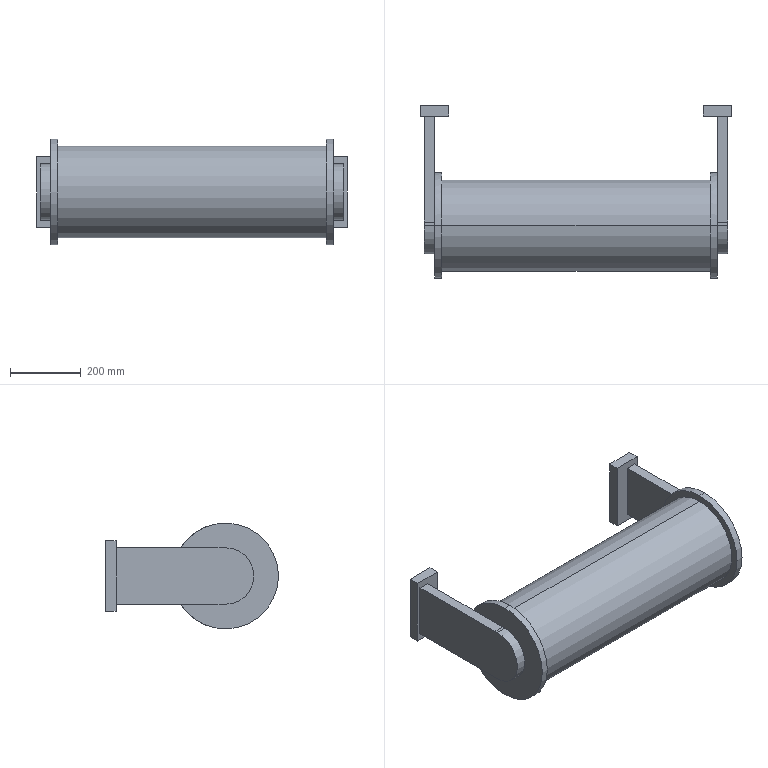Component | SolidWorks | LiftingAndOperatingMechanism-1_22-1 | 1 solid | 36 faces | box 880 x 490 x 300 mm | volume 47705868 mm3 | plane 24 | cylinder 12 | commonest cylinder face diameters 160 x6 300 x4 260 x2
build123d program:
from build123d import *

# Parameters (mm, degrees)
SKETCH3_R           = 150
BOSS_EXTRUDE1_DEPTH = 400
BOSS_EXTRUDE2_DEPTH = 30
SKETCH1_W           = 200
SKETCH1_H           = 80
BOSS_EXTRUDE3_DEPTH = 30
SKETCH5_R           = 150
SKETCH5_R_2         = 130
CUT_EXTRUDE1_DEPTH  = 380


with BuildPart() as part:
    # Sketch3 → Boss-Extrude1 (new, symmetric)
    with BuildSketch(Plane.XY):
        with Locations((0, 310)):
            Circle(SKETCH3_R)
    extrude(amount=BOSS_EXTRUDE1_DEPTH, both=True)

    # Sketch4 → Boss-Extrude2 (add)
    with BuildSketch(Plane.XY.offset(400)):
        with BuildLine():
            Line((-80, 0), (-79.382, 300.077))
            ThreePointArc((-79.382, 300.077), (0, 390), (79.382, 300.077))
            Line((79.382, 300.077), (80, 0))
            Line((80, 0), (-80, 0))
        make_face()
    boss_extrude2 = extrude(amount=BOSS_EXTRUDE2_DEPTH)

    # Mirror1: Boss-Extrude2 across plane
    add(boss_extrude2.mirror(Plane.XY))

    # Sketch1 → Boss-Extrude3 (add)
    with BuildSketch(Plane(origin=(0, 0, 0), x_dir=(1, 0, 0), z_dir=(0, 1, 0))):
        with Locations((0, 400)):
            Rectangle(SKETCH1_W, SKETCH1_H)
        with Locations((0, -400)):
            Rectangle(SKETCH1_W, SKETCH1_H)
    extrude(amount=-BOSS_EXTRUDE3_DEPTH)

    # Sketch5 → Cut-Extrude1 (cut, symmetric)
    with BuildSketch(Plane.XY):
        with Locations(Location((0, 310, 0), (0, 0, 237.939))):
            Circle(SKETCH5_R)
        with Locations((0, 310)):
            Circle(SKETCH5_R_2, mode=Mode.SUBTRACT)
    extrude(amount=CUT_EXTRUDE1_DEPTH, both=True, mode=Mode.SUBTRACT)


solid = part.part

# Placed as in the assembly
solid = solid.moved(Location((-1158.963, 12408.918, 7532.153), (180, 90, 0)))
STEP:
#1=COLOUR_RGB('',0.7922,0.8196,0.9333);
#2=FILL_AREA_STYLE_COLOUR('',#1);
#3=FILL_AREA_STYLE('',(#2));
#4=SURFACE_STYLE_FILL_AREA(#3);
#5=SURFACE_SIDE_STYLE('',(#4));
#6=SURFACE_STYLE_USAGE(.BOTH.,#5);
#7=PRESENTATION_STYLE_ASSIGNMENT((#6));
#8=CARTESIAN_POINT('',(-61.376,476.335,290.636));
#9=VERTEX_POINT('',#8);
#10=CARTESIAN_POINT('',(-61.376,476.335,302.447));
#11=VERTEX_POINT('',#10);
#12=CARTESIAN_POINT('',(-61.376,476.335,296.541));
#13=DIRECTION('',(-1.,-0.,0.0000002));
#14=DIRECTION('',(-0.0000002,0.,-1.));
#15=AXIS2_PLACEMENT_3D('',#12,#13,#14);
#16=CIRCLE('',#15,5.906);
#17=EDGE_CURVE('',#9,#11,#16,.T.);
#18=ORIENTED_EDGE('',*,*,#17,.F.);
#19=CARTESIAN_POINT('',(-60.589,476.335,290.636));
#20=VERTEX_POINT('',#19);
#21=CARTESIAN_POINT('',(-61.376,476.335,290.636));
#22=DIRECTION('',(1.,0.,-0.0000002));
#23=VECTOR('',#22,39.37);
#24=LINE('',#21,#23);
#25=EDGE_CURVE('',#9,#20,#24,.T.);
#26=ORIENTED_EDGE('',*,*,#25,.T.);
#27=CARTESIAN_POINT('',(-60.589,476.335,302.447));
#28=VERTEX_POINT('',#27);
#29=CARTESIAN_POINT('',(-60.589,476.335,296.541));
#30=DIRECTION('',(-1.,-0.,0.0000002));
#31=DIRECTION('',(-0.0000002,0.,-1.));
#32=AXIS2_PLACEMENT_3D('',#29,#30,#31);
#33=CIRCLE('',#32,5.906);
#34=EDGE_CURVE('',#20,#28,#33,.T.);
#35=ORIENTED_EDGE('',*,*,#34,.T.);
#36=CARTESIAN_POINT('',(-61.376,476.335,302.447));
#37=DIRECTION('',(1.,0.,-0.0000002));
#38=VECTOR('',#37,39.37);
#39=LINE('',#36,#38);
#40=EDGE_CURVE('',#11,#28,#39,.T.);
#41=ORIENTED_EDGE('',*,*,#40,.F.);
#42=EDGE_LOOP('',(#18,#26,#35,#41));
#43=FACE_OUTER_BOUND('',#42,.T.);
#44=CARTESIAN_POINT('',(-61.376,476.335,296.541));
#45=DIRECTION('',(1.,0.,-0.0000002));
#46=DIRECTION('',(0.0000002,0.,1.));
#47=AXIS2_PLACEMENT_3D('',#44,#45,#46);
#48=CYLINDRICAL_SURFACE('',#47,5.906);
#49=ADVANCED_FACE('',(#43),#48,.T.);
#50=CARTESIAN_POINT('',(-62.558,476.335,293.392));
#51=VERTEX_POINT('',#50);
#52=CARTESIAN_POINT('',(-62.558,476.335,299.691));
#53=VERTEX_POINT('',#52);
#54=CARTESIAN_POINT('',(-62.558,476.335,296.541));
#55=DIRECTION('',(-1.,-0.,0.0000002));
#56=DIRECTION('',(-0.0000002,0.,-1.));
#57=AXIS2_PLACEMENT_3D('',#54,#55,#56);
#58=CIRCLE('',#57,3.15);
#59=EDGE_CURVE('',#51,#53,#58,.T.);
#60=ORIENTED_EDGE('',*,*,#59,.F.);
#61=CARTESIAN_POINT('',(-61.376,476.335,293.392));
#62=VERTEX_POINT('',#61);
#63=CARTESIAN_POINT('',(-62.558,476.335,293.392));
#64=DIRECTION('',(1.,0.,-0.0000002));
#65=VECTOR('',#64,39.37);
#66=LINE('',#63,#65);
#67=EDGE_CURVE('',#51,#62,#66,.T.);
#68=ORIENTED_EDGE('',*,*,#67,.T.);
#69=CARTESIAN_POINT('',(-61.376,476.335,299.691));
#70=VERTEX_POINT('',#69);
#71=CARTESIAN_POINT('',(-61.376,476.335,296.541));
#72=DIRECTION('',(-1.,-0.,0.0000002));
#73=DIRECTION('',(-0.0000002,0.,-1.));
#74=AXIS2_PLACEMENT_3D('',#71,#72,#73);
#75=CIRCLE('',#74,3.15);
#76=EDGE_CURVE('',#62,#70,#75,.T.);
#77=ORIENTED_EDGE('',*,*,#76,.T.);
#78=CARTESIAN_POINT('',(-62.558,476.335,299.691));
#79=DIRECTION('',(1.,0.,-0.0000002));
#80=VECTOR('',#79,39.37);
#81=LINE('',#78,#80);
#82=EDGE_CURVE('',#53,#70,#81,.T.);
#83=ORIENTED_EDGE('',*,*,#82,.F.);
#84=EDGE_LOOP('',(#60,#68,#77,#83));
#85=FACE_OUTER_BOUND('',#84,.T.);
#86=CARTESIAN_POINT('',(-62.558,476.335,296.541));
#87=DIRECTION('',(1.,0.,-0.0000002));
#88=DIRECTION('',(0.0000002,0.,1.));
#89=AXIS2_PLACEMENT_3D('',#86,#87,#88);
#90=CYLINDRICAL_SURFACE('',#89,3.15);
#91=ADVANCED_FACE('',(#85),#90,.T.);
#92=CARTESIAN_POINT('',(-62.558,476.726,299.667));
#93=VERTEX_POINT('',#92);
#94=CARTESIAN_POINT('',(-62.558,476.335,296.541));
#95=DIRECTION('',(-1.,-0.,0.0000002));
#96=DIRECTION('',(-0.0000002,0.,-1.));
#97=AXIS2_PLACEMENT_3D('',#94,#95,#96);
#98=CIRCLE('',#97,3.15);
#99=EDGE_CURVE('',#53,#93,#98,.T.);
#100=ORIENTED_EDGE('',*,*,#99,.F.);
#101=ORIENTED_EDGE('',*,*,#82,.T.);
#102=CARTESIAN_POINT('',(-61.376,476.726,299.667));
#103=VERTEX_POINT('',#102);
#104=CARTESIAN_POINT('',(-61.376,476.335,296.541));
#105=DIRECTION('',(-1.,-0.,0.0000002));
#106=DIRECTION('',(-0.0000002,0.,-1.));
#107=AXIS2_PLACEMENT_3D('',#104,#105,#106);
#108=CIRCLE('',#107,3.15);
#109=EDGE_CURVE('',#70,#103,#108,.T.);
#110=ORIENTED_EDGE('',*,*,#109,.T.);
#111=CARTESIAN_POINT('',(-62.558,476.726,299.667));
#112=DIRECTION('',(1.,0.,-0.0000002));
#113=VECTOR('',#112,39.37);
#114=LINE('',#111,#113);
#115=EDGE_CURVE('',#93,#103,#114,.T.);
#116=ORIENTED_EDGE('',*,*,#115,.F.);
#117=EDGE_LOOP('',(#100,#101,#110,#116));
#118=FACE_OUTER_BOUND('',#117,.T.);
#119=CARTESIAN_POINT('',(-62.558,476.335,296.541));
#120=DIRECTION('',(1.,0.,-0.0000002));
#121=DIRECTION('',(0.0000002,0.,1.));
#122=AXIS2_PLACEMENT_3D('',#119,#120,#121);
#123=CYLINDRICAL_SURFACE('',#122,3.15);
#124=ADVANCED_FACE('',(#118),#123,.T.);
#125=CARTESIAN_POINT('',(-30.668,476.335,291.423));
#126=VERTEX_POINT('',#125);
#127=CARTESIAN_POINT('',(-30.668,476.335,301.66));
#128=VERTEX_POINT('',#127);
#129=CARTESIAN_POINT('',(-30.668,476.335,296.541));
#130=DIRECTION('',(-1.,-0.,0.0000002));
#131=DIRECTION('',(-0.0000002,0.,-1.));
#132=AXIS2_PLACEMENT_3D('',#129,#130,#131);
#133=CIRCLE('',#132,5.118);
#134=EDGE_CURVE('',#126,#128,#133,.T.);
#135=ORIENTED_EDGE('',*,*,#134,.T.);
#136=CARTESIAN_POINT('',(-60.589,476.335,301.66));
#137=VERTEX_POINT('',#136);
#138=CARTESIAN_POINT('',(-30.668,476.335,301.66));
#139=DIRECTION('',(-1.,-0.,0.0000002));
#140=VECTOR('',#139,39.37);
#141=LINE('',#138,#140);
#142=EDGE_CURVE('',#128,#137,#141,.T.);
#143=ORIENTED_EDGE('',*,*,#142,.T.);
#144=CARTESIAN_POINT('',(-60.589,476.335,291.423));
#145=VERTEX_POINT('',#144);
#146=CARTESIAN_POINT('',(-60.589,476.335,296.541));
#147=DIRECTION('',(-1.,-0.,0.0000002));
#148=DIRECTION('',(-0.0000002,0.,-1.));
#149=AXIS2_PLACEMENT_3D('',#146,#147,#148);
#150=CIRCLE('',#149,5.118);
#151=EDGE_CURVE('',#145,#137,#150,.T.);
#152=ORIENTED_EDGE('',*,*,#151,.F.);
#153=CARTESIAN_POINT('',(-30.668,476.335,291.423));
#154=DIRECTION('',(-1.,-0.,0.0000002));
#155=VECTOR('',#154,39.37);
#156=LINE('',#153,#155);
#157=EDGE_CURVE('',#126,#145,#156,.T.);
#158=ORIENTED_EDGE('',*,*,#157,.F.);
#159=EDGE_LOOP('',(#135,#143,#152,#158));
#160=FACE_OUTER_BOUND('',#159,.T.);
#161=CARTESIAN_POINT('',(-30.668,476.335,296.541));
#162=DIRECTION('',(-1.,-0.,0.0000002));
#163=DIRECTION('',(-0.0000002,0.,-1.));
#164=AXIS2_PLACEMENT_3D('',#161,#162,#163);
#165=CYLINDRICAL_SURFACE('',#164,5.118);
#166=ADVANCED_FACE('',(#160),#165,.T.);
#167=CARTESIAN_POINT('',(-28.699,476.335,293.392));
#168=VERTEX_POINT('',#167);
#169=CARTESIAN_POINT('',(-28.699,476.335,299.691));
#170=VERTEX_POINT('',#169);
#171=CARTESIAN_POINT('',(-28.699,476.335,296.541));
#172=DIRECTION('',(-1.,-0.,0.0000002));
#173=DIRECTION('',(-0.0000002,0.,-1.));
#174=AXIS2_PLACEMENT_3D('',#171,#172,#173);
#175=CIRCLE('',#174,3.15);
#176=EDGE_CURVE('',#168,#170,#175,.T.);
#177=ORIENTED_EDGE('',*,*,#176,.T.);
#178=CARTESIAN_POINT('',(-29.88,476.335,299.691));
#179=VERTEX_POINT('',#178);
#180=CARTESIAN_POINT('',(-28.699,476.335,299.691));
#181=DIRECTION('',(-1.,-0.,0.0000002));
#182=VECTOR('',#181,39.37);
#183=LINE('',#180,#182);
#184=EDGE_CURVE('',#170,#179,#183,.T.);
#185=ORIENTED_EDGE('',*,*,#184,.T.);
#186=CARTESIAN_POINT('',(-29.88,476.335,293.392));
#187=VERTEX_POINT('',#186);
#188=CARTESIAN_POINT('',(-29.88,476.335,296.541));
#189=DIRECTION('',(-1.,-0.,0.0000002));
#190=DIRECTION('',(-0.0000002,0.,-1.));
#191=AXIS2_PLACEMENT_3D('',#188,#189,#190);
#192=CIRCLE('',#191,3.15);
#193=EDGE_CURVE('',#187,#179,#192,.T.);
#194=ORIENTED_EDGE('',*,*,#193,.F.);
#195=CARTESIAN_POINT('',(-28.699,476.335,293.392));
#196=DIRECTION('',(-1.,-0.,0.0000002));
#197=VECTOR('',#196,39.37);
#198=LINE('',#195,#197);
#199=EDGE_CURVE('',#168,#187,#198,.T.);
#200=ORIENTED_EDGE('',*,*,#199,.F.);
#201=EDGE_LOOP('',(#177,#185,#194,#200));
#202=FACE_OUTER_BOUND('',#201,.T.);
#203=CARTESIAN_POINT('',(-28.699,476.335,296.541));
#204=DIRECTION('',(-1.,-0.,0.0000002));
#205=DIRECTION('',(-0.0000002,0.,-1.));
#206=AXIS2_PLACEMENT_3D('',#203,#204,#205);
#207=CYLINDRICAL_SURFACE('',#206,3.15);
#208=ADVANCED_FACE('',(#202),#207,.T.);
#209=CARTESIAN_POINT('',(-28.699,476.726,293.416));
#210=VERTEX_POINT('',#209);
#211=CARTESIAN_POINT('',(-28.699,476.335,296.541));
#212=DIRECTION('',(-1.,-0.,0.0000002));
#213=DIRECTION('',(-0.0000002,0.,-1.));
#214=AXIS2_PLACEMENT_3D('',#211,#212,#213);
#215=CIRCLE('',#214,3.15);
#216=EDGE_CURVE('',#210,#168,#215,.T.);
#217=ORIENTED_EDGE('',*,*,#216,.T.);
#218=ORIENTED_EDGE('',*,*,#199,.T.);
#219=CARTESIAN_POINT('',(-29.88,476.726,293.416));
#220=VERTEX_POINT('',#219);
#221=CARTESIAN_POINT('',(-29.88,476.335,296.541));
#222=DIRECTION('',(-1.,-0.,0.0000002));
#223=DIRECTION('',(-0.0000002,0.,-1.));
#224=AXIS2_PLACEMENT_3D('',#221,#222,#223);
#225=CIRCLE('',#224,3.15);
#226=EDGE_CURVE('',#220,#187,#225,.T.);
#227=ORIENTED_EDGE('',*,*,#226,.F.);
#228=CARTESIAN_POINT('',(-28.699,476.726,293.416));
#229=DIRECTION('',(-1.,-0.,0.0000002));
#230=VECTOR('',#229,39.37);
#231=LINE('',#228,#230);
#232=EDGE_CURVE('',#210,#220,#231,.T.);
#233=ORIENTED_EDGE('',*,*,#232,.F.);
#234=EDGE_LOOP('',(#217,#218,#227,#233));
#235=FACE_OUTER_BOUND('',#234,.T.);
#236=CARTESIAN_POINT('',(-28.699,476.335,296.541));
#237=DIRECTION('',(-1.,-0.,0.0000002));
#238=DIRECTION('',(-0.0000002,0.,-1.));
#239=AXIS2_PLACEMENT_3D('',#236,#237,#238);
#240=CYLINDRICAL_SURFACE('',#239,3.15);
#241=ADVANCED_FACE('',(#235),#240,.T.);
#242=CARTESIAN_POINT('',(-30.668,476.335,290.636));
#243=VERTEX_POINT('',#242);
#244=CARTESIAN_POINT('',(-30.668,476.335,302.447));
#245=VERTEX_POINT('',#244);
#246=CARTESIAN_POINT('',(-30.668,476.335,296.541));
#247=DIRECTION('',(-1.,-0.,0.0000002));
#248=DIRECTION('',(-0.0000002,0.,-1.));
#249=AXIS2_PLACEMENT_3D('',#246,#247,#248);
#250=CIRCLE('',#249,5.906);
#251=EDGE_CURVE('',#243,#245,#250,.T.);
#252=ORIENTED_EDGE('',*,*,#251,.F.);
#253=CARTESIAN_POINT('',(-29.88,476.335,290.636));
#254=VERTEX_POINT('',#253);
#255=CARTESIAN_POINT('',(-61.376,476.335,290.636));
#256=DIRECTION('',(1.,0.,-0.0000002));
#257=VECTOR('',#256,39.37);
#258=LINE('',#255,#257);
#259=EDGE_CURVE('',#243,#254,#258,.T.);
#260=ORIENTED_EDGE('',*,*,#259,.T.);
#261=CARTESIAN_POINT('',(-29.88,476.335,302.447));
#262=VERTEX_POINT('',#261);
#263=CARTESIAN_POINT('',(-29.88,476.335,296.541));
#264=DIRECTION('',(-1.,-0.,0.0000002));
#265=DIRECTION('',(-0.0000002,0.,-1.));
#266=AXIS2_PLACEMENT_3D('',#263,#264,#265);
#267=CIRCLE('',#266,5.906);
#268=EDGE_CURVE('',#254,#262,#267,.T.);
#269=ORIENTED_EDGE('',*,*,#268,.T.);
#270=CARTESIAN_POINT('',(-61.376,476.335,302.447));
#271=DIRECTION('',(1.,0.,-0.0000002));
#272=VECTOR('',#271,39.37);
#273=LINE('',#270,#272);
#274=EDGE_CURVE('',#245,#262,#273,.T.);
#275=ORIENTED_EDGE('',*,*,#274,.F.);
#276=EDGE_LOOP('',(#252,#260,#269,#275));
#277=FACE_OUTER_BOUND('',#276,.T.);
#278=CARTESIAN_POINT('',(-61.376,476.335,296.541));
#279=DIRECTION('',(1.,0.,-0.0000002));
#280=DIRECTION('',(0.0000002,0.,1.));
#281=AXIS2_PLACEMENT_3D('',#278,#279,#280);
#282=CYLINDRICAL_SURFACE('',#281,5.906);
#283=ADVANCED_FACE('',(#277),#282,.T.);
#284=ORIENTED_EDGE('',*,*,#259,.F.);
#285=CARTESIAN_POINT('',(-30.668,476.335,296.541));
#286=DIRECTION('',(-1.,-0.,0.0000002));
#287=DIRECTION('',(-0.0000002,0.,-1.));
#288=AXIS2_PLACEMENT_3D('',#285,#286,#287);
#289=CIRCLE('',#288,5.906);
#290=EDGE_CURVE('',#245,#243,#289,.T.);
#291=ORIENTED_EDGE('',*,*,#290,.F.);
#292=ORIENTED_EDGE('',*,*,#274,.T.);
#293=CARTESIAN_POINT('',(-29.88,481.34,299.676));
#294=VERTEX_POINT('',#293);
#295=CARTESIAN_POINT('',(-29.88,476.335,296.541));
#296=DIRECTION('',(-1.,-0.,0.0000002));
#297=DIRECTION('',(-0.0000002,0.,-1.));
#298=AXIS2_PLACEMENT_3D('',#295,#296,#297);
#299=CIRCLE('',#298,5.906);
#300=EDGE_CURVE('',#262,#294,#299,.T.);
#301=ORIENTED_EDGE('',*,*,#300,.T.);
#302=CARTESIAN_POINT('',(-29.88,481.34,293.407));
#303=VERTEX_POINT('',#302);
#304=CARTESIAN_POINT('',(-29.88,476.335,296.541));
#305=DIRECTION('',(-1.,-0.,0.0000002));
#306=DIRECTION('',(-0.0000002,0.,-1.));
#307=AXIS2_PLACEMENT_3D('',#304,#305,#306);
#308=CIRCLE('',#307,5.906);
#309=EDGE_CURVE('',#294,#303,#308,.T.);
#310=ORIENTED_EDGE('',*,*,#309,.T.);
#311=CARTESIAN_POINT('',(-29.88,476.335,296.541));
#312=DIRECTION('',(-1.,-0.,0.0000002));
#313=DIRECTION('',(-0.0000002,0.,-1.));
#314=AXIS2_PLACEMENT_3D('',#311,#312,#313);
#315=CIRCLE('',#314,5.906);
#316=EDGE_CURVE('',#303,#254,#315,.T.);
#317=ORIENTED_EDGE('',*,*,#316,.T.);
#318=EDGE_LOOP('',(#284,#291,#292,#301,#310,#317));
#319=FACE_OUTER_BOUND('',#318,.T.);
#320=CARTESIAN_POINT('',(-61.376,476.335,296.541));
#321=DIRECTION('',(1.,0.,-0.0000002));
#322=DIRECTION('',(0.0000002,0.,1.));
#323=AXIS2_PLACEMENT_3D('',#320,#321,#322);
#324=CYLINDRICAL_SURFACE('',#323,5.906);
#325=ADVANCED_FACE('',(#319),#324,.T.);
#326=ORIENTED_EDGE('',*,*,#316,.F.);
#327=CARTESIAN_POINT('',(-29.88,488.54,293.392));
#328=DIRECTION('',(0.,-1.,0.002059));
#329=VECTOR('',#328,39.37);
#330=LINE('',#327,#329);
#331=EDGE_CURVE('',#303,#220,#330,.T.);
#332=ORIENTED_EDGE('',*,*,#331,.T.);
#333=ORIENTED_EDGE('',*,*,#226,.T.);
#334=ORIENTED_EDGE('',*,*,#193,.T.);
#335=CARTESIAN_POINT('',(-29.88,476.726,299.667));
#336=VERTEX_POINT('',#335);
#337=CARTESIAN_POINT('',(-29.88,476.335,296.541));
#338=DIRECTION('',(-1.,-0.,0.0000002));
#339=DIRECTION('',(-0.0000002,0.,-1.));
#340=AXIS2_PLACEMENT_3D('',#337,#338,#339);
#341=CIRCLE('',#340,3.15);
#342=EDGE_CURVE('',#179,#336,#341,.T.);
#343=ORIENTED_EDGE('',*,*,#342,.T.);
#344=CARTESIAN_POINT('',(-29.88,488.54,299.691));
#345=DIRECTION('',(0.,1.,0.002059));
#346=VECTOR('',#345,39.37);
#347=LINE('',#344,#346);
#348=EDGE_CURVE('',#336,#294,#347,.T.);
#349=ORIENTED_EDGE('',*,*,#348,.T.);
#350=ORIENTED_EDGE('',*,*,#300,.F.);
#351=ORIENTED_EDGE('',*,*,#268,.F.);
#352=EDGE_LOOP('',(#326,#332,#333,#334,#343,#349,#350,#351));
#353=FACE_OUTER_BOUND('',#352,.T.);
#354=CARTESIAN_POINT('',(-29.88,476.335,296.541));
#355=DIRECTION('',(-1.,-0.,0.0000002));
#356=DIRECTION('',(-0.0000002,0.,-1.));
#357=AXIS2_PLACEMENT_3D('',#354,#355,#356);
#358=PLANE('',#357);
#359=ADVANCED_FACE('',(#353),#358,.F.);
#360=ORIENTED_EDGE('',*,*,#348,.F.);
#361=CARTESIAN_POINT('',(-28.699,476.726,299.667));
#362=VERTEX_POINT('',#361);
#363=CARTESIAN_POINT('',(-28.699,476.726,299.667));
#364=DIRECTION('',(-1.,-0.,0.0000002));
#365=VECTOR('',#364,39.37);
#366=LINE('',#363,#365);
#367=EDGE_CURVE('',#362,#336,#366,.T.);
#368=ORIENTED_EDGE('',*,*,#367,.F.);
#369=CARTESIAN_POINT('',(-28.699,488.54,299.691));
#370=VERTEX_POINT('',#369);
#371=CARTESIAN_POINT('',(-28.699,488.54,299.691));
#372=DIRECTION('',(0.,1.,0.002059));
#373=VECTOR('',#372,39.37);
#374=LINE('',#371,#373);
#375=EDGE_CURVE('',#362,#370,#374,.T.);
#376=ORIENTED_EDGE('',*,*,#375,.T.);
#377=CARTESIAN_POINT('',(-29.88,488.54,299.691));
#378=VERTEX_POINT('',#377);
#379=CARTESIAN_POINT('',(-28.699,488.54,299.691));
#380=DIRECTION('',(-1.,-0.,0.0000002));
#381=VECTOR('',#380,39.37);
#382=LINE('',#379,#381);
#383=EDGE_CURVE('',#370,#378,#382,.T.);
#384=ORIENTED_EDGE('',*,*,#383,.T.);
#385=CARTESIAN_POINT('',(-29.88,488.54,299.691));
#386=DIRECTION('',(0.,1.,0.002059));
#387=VECTOR('',#386,39.37);
#388=LINE('',#385,#387);
#389=EDGE_CURVE('',#294,#378,#388,.T.);
#390=ORIENTED_EDGE('',*,*,#389,.F.);
#391=EDGE_LOOP('',(#360,#368,#376,#384,#390));
#392=FACE_OUTER_BOUND('',#391,.T.);
#393=CARTESIAN_POINT('',(-28.699,488.54,299.691));
#394=DIRECTION('',(0.0000002,-0.002059,1.));
#395=DIRECTION('',(0.,1.,0.002059));
#396=AXIS2_PLACEMENT_3D('',#393,#394,#395);
#397=PLANE('',#396);
#398=ADVANCED_FACE('',(#392),#397,.T.);
#399=ORIENTED_EDGE('',*,*,#184,.F.);
#400=CARTESIAN_POINT('',(-28.699,476.335,296.541));
#401=DIRECTION('',(-1.,-0.,0.0000002));
#402=DIRECTION('',(-0.0000002,0.,-1.));
#403=AXIS2_PLACEMENT_3D('',#400,#401,#402);
#404=CIRCLE('',#403,3.15);
#405=EDGE_CURVE('',#170,#362,#404,.T.);
#406=ORIENTED_EDGE('',*,*,#405,.T.);
#407=ORIENTED_EDGE('',*,*,#367,.T.);
#408=ORIENTED_EDGE('',*,*,#342,.F.);
#409=EDGE_LOOP('',(#399,#406,#407,#408));
#410=FACE_OUTER_BOUND('',#409,.T.);
#411=CARTESIAN_POINT('',(-28.699,476.335,296.541));
#412=DIRECTION('',(-1.,-0.,0.0000002));
#413=DIRECTION('',(-0.0000002,0.,-1.));
#414=AXIS2_PLACEMENT_3D('',#411,#412,#413);
#415=CYLINDRICAL_SURFACE('',#414,3.15);
#416=ADVANCED_FACE('',(#410),#415,.T.);
#417=CARTESIAN_POINT('',(-29.88,488.54,293.392));
#418=VERTEX_POINT('',#417);
#419=CARTESIAN_POINT('',(-29.88,488.54,293.392));
#420=DIRECTION('',(0.,-1.,0.002059));
#421=VECTOR('',#420,39.37);
#422=LINE('',#419,#421);
#423=EDGE_CURVE('',#418,#303,#422,.T.);
#424=ORIENTED_EDGE('',*,*,#423,.F.);
#425=CARTESIAN_POINT('',(-28.699,488.54,293.392));
#426=VERTEX_POINT('',#425);
#427=CARTESIAN_POINT('',(-28.699,488.54,293.392));
#428=DIRECTION('',(-1.,-0.,0.0000002));
#429=VECTOR('',#428,39.37);
#430=LINE('',#427,#429);
#431=EDGE_CURVE('',#426,#418,#430,.T.);
#432=ORIENTED_EDGE('',*,*,#431,.F.);
#433=CARTESIAN_POINT('',(-28.699,488.54,293.392));
#434=DIRECTION('',(0.,-1.,0.002059));
#435=VECTOR('',#434,39.37);
#436=LINE('',#433,#435);
#437=EDGE_CURVE('',#426,#210,#436,.T.);
#438=ORIENTED_EDGE('',*,*,#437,.T.);
#439=ORIENTED_EDGE('',*,*,#232,.T.);
#440=ORIENTED_EDGE('',*,*,#331,.F.);
#441=EDGE_LOOP('',(#424,#432,#438,#439,#440));
#442=FACE_OUTER_BOUND('',#441,.T.);
#443=CARTESIAN_POINT('',(-28.699,488.54,293.392));
#444=DIRECTION('',(-0.0000002,-0.002059,-1.));
#445=DIRECTION('',(0.,-1.,0.002059));
#446=AXIS2_PLACEMENT_3D('',#443,#444,#445);
#447=PLANE('',#446);
#448=ADVANCED_FACE('',(#442),#447,.T.);
#449=CARTESIAN_POINT('',(-28.699,488.54,299.691));
#450=DIRECTION('',(-0.0000002,0.,-1.));
#451=VECTOR('',#450,39.37);
#452=LINE('',#449,#451);
#453=EDGE_CURVE('',#370,#426,#452,.T.);
#454=ORIENTED_EDGE('',*,*,#453,.F.);
#455=ORIENTED_EDGE('',*,*,#375,.F.);
#456=ORIENTED_EDGE('',*,*,#405,.F.);
#457=ORIENTED_EDGE('',*,*,#176,.F.);
#458=ORIENTED_EDGE('',*,*,#216,.F.);
#459=ORIENTED_EDGE('',*,*,#437,.F.);
#460=EDGE_LOOP('',(#454,#455,#456,#457,#458,#459));
#461=FACE_OUTER_BOUND('',#460,.T.);
#462=CARTESIAN_POINT('',(-28.699,476.335,296.541));
#463=DIRECTION('',(1.,0.,-0.0000002));
#464=DIRECTION('',(-0.0000002,0.,-1.));
#465=AXIS2_PLACEMENT_3D('',#462,#463,#464);
#466=PLANE('',#465);
#467=ADVANCED_FACE('',(#461),#466,.T.);
#468=ORIENTED_EDGE('',*,*,#309,.F.);
#469=ORIENTED_EDGE('',*,*,#389,.T.);
#470=CARTESIAN_POINT('',(-29.88,488.54,299.691));
#471=DIRECTION('',(-0.0000002,0.,-1.));
#472=VECTOR('',#471,39.37);
#473=LINE('',#470,#472);
#474=EDGE_CURVE('',#378,#418,#473,.T.);
#475=ORIENTED_EDGE('',*,*,#474,.T.);
#476=ORIENTED_EDGE('',*,*,#423,.T.);
#477=EDGE_LOOP('',(#468,#469,#475,#476));
#478=FACE_OUTER_BOUND('',#477,.T.);
#479=CARTESIAN_POINT('',(-29.88,476.335,296.541));
#480=DIRECTION('',(1.,0.,-0.0000002));
#481=DIRECTION('',(-0.0000002,0.,-1.));
#482=AXIS2_PLACEMENT_3D('',#479,#480,#481);
#483=PLANE('',#482);
#484=ADVANCED_FACE('',(#478),#483,.F.);
#485=CARTESIAN_POINT('',(-31.455,488.54,292.604));
#486=VERTEX_POINT('',#485);
#487=CARTESIAN_POINT('',(-28.306,488.54,292.604));
#488=VERTEX_POINT('',#487);
#489=CARTESIAN_POINT('',(-28.306,488.54,292.604));
#490=DIRECTION('',(1.,0.,-0.0000002));
#491=VECTOR('',#490,39.37);
#492=LINE('',#489,#491);
#493=EDGE_CURVE('',#486,#488,#492,.T.);
#494=ORIENTED_EDGE('',*,*,#493,.T.);
#495=CARTESIAN_POINT('',(-28.306,488.54,300.478));
#496=VERTEX_POINT('',#495);
#497=CARTESIAN_POINT('',(-28.306,488.54,300.478));
#498=DIRECTION('',(0.0000002,-0.,1.));
#499=VECTOR('',#498,39.37);
#500=LINE('',#497,#499);
#501=EDGE_CURVE('',#488,#496,#500,.T.);
#502=ORIENTED_EDGE('',*,*,#501,.T.);
#503=CARTESIAN_POINT('',(-31.455,488.54,300.478));
#504=VERTEX_POINT('',#503);
#505=CARTESIAN_POINT('',(-28.306,488.54,300.478));
#506=DIRECTION('',(-1.,-0.,0.0000002));
#507=VECTOR('',#506,39.37);
#508=LINE('',#505,#507);
#509=EDGE_CURVE('',#496,#504,#508,.T.);
#510=ORIENTED_EDGE('',*,*,#509,.T.);
#511=CARTESIAN_POINT('',(-31.455,488.54,300.478));
#512=DIRECTION('',(-0.0000002,0.,-1.));
#513=VECTOR('',#512,39.37);
#514=LINE('',#511,#513);
#515=EDGE_CURVE('',#504,#486,#514,.T.);
#516=ORIENTED_EDGE('',*,*,#515,.T.);
#517=EDGE_LOOP('',(#494,#502,#510,#516));
#518=FACE_OUTER_BOUND('',#517,.T.);
#519=ORIENTED_EDGE('',*,*,#474,.F.);
#520=ORIENTED_EDGE('',*,*,#383,.F.);
#521=ORIENTED_EDGE('',*,*,#453,.T.);
#522=ORIENTED_EDGE('',*,*,#431,.T.);
#523=EDGE_LOOP('',(#519,#520,#521,#522));
#524=FACE_BOUND('',#523,.T.);
#525=CARTESIAN_POINT('',(-45.628,488.54,296.541));
#526=DIRECTION('',(0.,-1.,-0.));
#527=DIRECTION('',(-1.,-0.,0.0000002));
#528=AXIS2_PLACEMENT_3D('',#525,#526,#527);
#529=PLANE('',#528);
#530=ADVANCED_FACE('',(#518,#524),#529,.T.);
#531=ORIENTED_EDGE('',*,*,#493,.F.);
#532=CARTESIAN_POINT('',(-31.455,489.721,292.604));
#533=VERTEX_POINT('',#532);
#534=CARTESIAN_POINT('',(-31.455,489.721,292.604));
#535=DIRECTION('',(0.,-1.,-0.));
#536=VECTOR('',#535,39.37);
#537=LINE('',#534,#536);
#538=EDGE_CURVE('',#533,#486,#537,.T.);
#539=ORIENTED_EDGE('',*,*,#538,.F.);
#540=CARTESIAN_POINT('',(-28.306,489.721,292.604));
#541=VERTEX_POINT('',#540);
#542=CARTESIAN_POINT('',(-28.306,489.721,292.604));
#543=DIRECTION('',(1.,0.,-0.0000002));
#544=VECTOR('',#543,39.37);
#545=LINE('',#542,#544);
#546=EDGE_CURVE('',#533,#541,#545,.T.);
#547=ORIENTED_EDGE('',*,*,#546,.T.);
#548=CARTESIAN_POINT('',(-28.306,489.721,292.604));
#549=DIRECTION('',(0.,-1.,-0.));
#550=VECTOR('',#549,39.37);
#551=LINE('',#548,#550);
#552=EDGE_CURVE('',#541,#488,#551,.T.);
#553=ORIENTED_EDGE('',*,*,#552,.T.);
#554=EDGE_LOOP('',(#531,#539,#547,#553));
#555=FACE_OUTER_BOUND('',#554,.T.);
#556=CARTESIAN_POINT('',(-28.306,489.721,292.604));
#557=DIRECTION('',(-0.0000002,0.,-1.));
#558=DIRECTION('',(1.,0.,-0.0000002));
#559=AXIS2_PLACEMENT_3D('',#556,#557,#558);
#560=PLANE('',#559);
#561=ADVANCED_FACE('',(#555),#560,.T.);
#562=ORIENTED_EDGE('',*,*,#515,.F.);
#563=CARTESIAN_POINT('',(-31.455,489.721,300.478));
#564=VERTEX_POINT('',#563);
#565=CARTESIAN_POINT('',(-31.455,489.721,300.478));
#566=DIRECTION('',(0.,-1.,-0.));
#567=VECTOR('',#566,39.37);
#568=LINE('',#565,#567);
#569=EDGE_CURVE('',#564,#504,#568,.T.);
#570=ORIENTED_EDGE('',*,*,#569,.F.);
#571=CARTESIAN_POINT('',(-31.455,489.721,300.478));
#572=DIRECTION('',(-0.0000002,0.,-1.));
#573=VECTOR('',#572,39.37);
#574=LINE('',#571,#573);
#575=EDGE_CURVE('',#564,#533,#574,.T.);
#576=ORIENTED_EDGE('',*,*,#575,.T.);
#577=ORIENTED_EDGE('',*,*,#538,.T.);
#578=EDGE_LOOP('',(#562,#570,#576,#577));
#579=FACE_OUTER_BOUND('',#578,.T.);
#580=CARTESIAN_POINT('',(-31.455,489.721,300.478));
#581=DIRECTION('',(-1.,-0.,0.0000002));
#582=DIRECTION('',(-0.0000002,0.,-1.));
#583=AXIS2_PLACEMENT_3D('',#580,#581,#582);
#584=PLANE('',#583);
#585=ADVANCED_FACE('',(#579),#584,.T.);
#586=ORIENTED_EDGE('',*,*,#509,.F.);
#587=CARTESIAN_POINT('',(-28.306,489.721,300.478));
#588=VERTEX_POINT('',#587);
#589=CARTESIAN_POINT('',(-28.306,489.721,300.478));
#590=DIRECTION('',(0.,-1.,-0.));
#591=VECTOR('',#590,39.37);
#592=LINE('',#589,#591);
#593=EDGE_CURVE('',#588,#496,#592,.T.);
#594=ORIENTED_EDGE('',*,*,#593,.F.);
#595=CARTESIAN_POINT('',(-28.306,489.721,300.478));
#596=DIRECTION('',(-1.,-0.,0.0000002));
#597=VECTOR('',#596,39.37);
#598=LINE('',#595,#597);
#599=EDGE_CURVE('',#588,#564,#598,.T.);
#600=ORIENTED_EDGE('',*,*,#599,.T.);
#601=ORIENTED_EDGE('',*,*,#569,.T.);
#602=EDGE_LOOP('',(#586,#594,#600,#601));
#603=FACE_OUTER_BOUND('',#602,.T.);
#604=CARTESIAN_POINT('',(-28.306,489.721,300.478));
#605=DIRECTION('',(0.0000002,-0.,1.));
#606=DIRECTION('',(-1.,-0.,0.0000002));
#607=AXIS2_PLACEMENT_3D('',#604,#605,#606);
#608=PLANE('',#607);
#609=ADVANCED_FACE('',(#603),#608,.T.);
#610=ORIENTED_EDGE('',*,*,#501,.F.);
#611=ORIENTED_EDGE('',*,*,#552,.F.);
#612=CARTESIAN_POINT('',(-28.306,489.721,300.478));
#613=DIRECTION('',(0.0000002,-0.,1.));
#614=VECTOR('',#613,39.37);
#615=LINE('',#612,#614);
#616=EDGE_CURVE('',#541,#588,#615,.T.);
#617=ORIENTED_EDGE('',*,*,#616,.T.);
#618=ORIENTED_EDGE('',*,*,#593,.T.);
#619=EDGE_LOOP('',(#610,#611,#617,#618));
#620=FACE_OUTER_BOUND('',#619,.T.);
#621=CARTESIAN_POINT('',(-28.306,489.721,300.478));
#622=DIRECTION('',(1.,0.,-0.0000002));
#623=DIRECTION('',(0.0000002,-0.,1.));
#624=AXIS2_PLACEMENT_3D('',#621,#622,#623);
#625=PLANE('',#624);
#626=ADVANCED_FACE('',(#620),#625,.T.);
#627=ORIENTED_EDGE('',*,*,#546,.F.);
#628=ORIENTED_EDGE('',*,*,#575,.F.);
#629=ORIENTED_EDGE('',*,*,#599,.F.);
#630=ORIENTED_EDGE('',*,*,#616,.F.);
#631=EDGE_LOOP('',(#627,#628,#629,#630));
#632=FACE_OUTER_BOUND('',#631,.T.);
#633=CARTESIAN_POINT('',(-45.628,489.721,296.541));
#634=DIRECTION('',(0.,-1.,-0.));
#635=DIRECTION('',(-1.,-0.,0.0000002));
#636=AXIS2_PLACEMENT_3D('',#633,#634,#635);
#637=PLANE('',#636);
#638=ADVANCED_FACE('',(#632),#637,.F.);
#639=ORIENTED_EDGE('',*,*,#134,.F.);
#640=CARTESIAN_POINT('',(-30.668,476.335,296.541));
#641=DIRECTION('',(-1.,-0.,0.0000002));
#642=DIRECTION('',(-0.0000002,0.,-1.));
#643=AXIS2_PLACEMENT_3D('',#640,#641,#642);
#644=CIRCLE('',#643,5.118);
#645=EDGE_CURVE('',#128,#126,#644,.T.);
#646=ORIENTED_EDGE('',*,*,#645,.F.);
#647=EDGE_LOOP('',(#639,#646));
#648=FACE_BOUND('',#647,.T.);
#649=ORIENTED_EDGE('',*,*,#290,.T.);
#650=ORIENTED_EDGE('',*,*,#251,.T.);
#651=EDGE_LOOP('',(#649,#650));
#652=FACE_OUTER_BOUND('',#651,.T.);
#653=CARTESIAN_POINT('',(-30.668,476.335,296.541));
#654=DIRECTION('',(-1.,-0.,0.0000002));
#655=DIRECTION('',(-0.0000002,0.,-1.));
#656=AXIS2_PLACEMENT_3D('',#653,#654,#655);
#657=PLANE('',#656);
#658=ADVANCED_FACE('',(#648,#652),#657,.T.);
#659=ORIENTED_EDGE('',*,*,#151,.T.);
#660=CARTESIAN_POINT('',(-60.589,476.335,296.541));
#661=DIRECTION('',(-1.,-0.,0.0000002));
#662=DIRECTION('',(-0.0000002,0.,-1.));
#663=AXIS2_PLACEMENT_3D('',#660,#661,#662);
#664=CIRCLE('',#663,5.118);
#665=EDGE_CURVE('',#137,#145,#664,.T.);
#666=ORIENTED_EDGE('',*,*,#665,.T.);
#667=EDGE_LOOP('',(#659,#666));
#668=FACE_BOUND('',#667,.T.);
#669=CARTESIAN_POINT('',(-60.589,476.335,296.541));
#670=DIRECTION('',(-1.,-0.,0.0000002));
#671=DIRECTION('',(-0.0000002,0.,-1.));
#672=AXIS2_PLACEMENT_3D('',#669,#670,#671);
#673=CIRCLE('',#672,5.906);
#674=EDGE_CURVE('',#28,#20,#673,.T.);
#675=ORIENTED_EDGE('',*,*,#674,.F.);
#676=ORIENTED_EDGE('',*,*,#34,.F.);
#677=EDGE_LOOP('',(#675,#676));
#678=FACE_OUTER_BOUND('',#677,.T.);
#679=CARTESIAN_POINT('',(-60.589,476.335,296.541));
#680=DIRECTION('',(-1.,-0.,0.0000002));
#681=DIRECTION('',(-0.0000002,0.,-1.));
#682=AXIS2_PLACEMENT_3D('',#679,#680,#681);
#683=PLANE('',#682);
#684=ADVANCED_FACE('',(#668,#678),#683,.F.);
#685=ORIENTED_EDGE('',*,*,#142,.F.);
#686=ORIENTED_EDGE('',*,*,#645,.T.);
#687=ORIENTED_EDGE('',*,*,#157,.T.);
#688=ORIENTED_EDGE('',*,*,#665,.F.);
#689=EDGE_LOOP('',(#685,#686,#687,#688));
#690=FACE_OUTER_BOUND('',#689,.T.);
#691=CARTESIAN_POINT('',(-30.668,476.335,296.541));
#692=DIRECTION('',(-1.,-0.,0.0000002));
#693=DIRECTION('',(-0.0000002,0.,-1.));
#694=AXIS2_PLACEMENT_3D('',#691,#692,#693);
#695=CYLINDRICAL_SURFACE('',#694,5.118);
#696=ADVANCED_FACE('',(#690),#695,.T.);
#697=CARTESIAN_POINT('',(-59.802,489.721,300.478));
#698=VERTEX_POINT('',#697);
#699=CARTESIAN_POINT('',(-62.951,489.721,300.478));
#700=VERTEX_POINT('',#699);
#701=CARTESIAN_POINT('',(-62.951,489.721,300.478));
#702=DIRECTION('',(-1.,-0.,0.0000002));
#703=VECTOR('',#702,39.37);
#704=LINE('',#701,#703);
#705=EDGE_CURVE('',#698,#700,#704,.T.);
#706=ORIENTED_EDGE('',*,*,#705,.F.);
#707=CARTESIAN_POINT('',(-59.802,489.721,292.604));
#708=VERTEX_POINT('',#707);
#709=CARTESIAN_POINT('',(-59.802,489.721,300.478));
#710=DIRECTION('',(0.0000002,-0.,1.));
#711=VECTOR('',#710,39.37);
#712=LINE('',#709,#711);
#713=EDGE_CURVE('',#708,#698,#712,.T.);
#714=ORIENTED_EDGE('',*,*,#713,.F.);
#715=CARTESIAN_POINT('',(-62.951,489.721,292.604));
#716=VERTEX_POINT('',#715);
#717=CARTESIAN_POINT('',(-62.951,489.721,292.604));
#718=DIRECTION('',(1.,0.,-0.0000002));
#719=VECTOR('',#718,39.37);
#720=LINE('',#717,#719);
#721=EDGE_CURVE('',#716,#708,#720,.T.);
#722=ORIENTED_EDGE('',*,*,#721,.F.);
#723=CARTESIAN_POINT('',(-62.951,489.721,300.478));
#724=DIRECTION('',(-0.0000002,0.,-1.));
#725=VECTOR('',#724,39.37);
#726=LINE('',#723,#725);
#727=EDGE_CURVE('',#700,#716,#726,.T.);
#728=ORIENTED_EDGE('',*,*,#727,.F.);
#729=EDGE_LOOP('',(#706,#714,#722,#728));
#730=FACE_OUTER_BOUND('',#729,.T.);
#731=CARTESIAN_POINT('',(-45.628,489.721,296.541));
#732=DIRECTION('',(-0.,1.,0.));
#733=DIRECTION('',(1.,0.,-0.0000002));
#734=AXIS2_PLACEMENT_3D('',#731,#732,#733);
#735=PLANE('',#734);
#736=ADVANCED_FACE('',(#730),#735,.T.);
#737=CARTESIAN_POINT('',(-59.802,488.54,292.604));
#738=VERTEX_POINT('',#737);
#739=CARTESIAN_POINT('',(-59.802,488.54,300.478));
#740=VERTEX_POINT('',#739);
#741=CARTESIAN_POINT('',(-59.802,488.54,300.478));
#742=DIRECTION('',(0.0000002,-0.,1.));
#743=VECTOR('',#742,39.37);
#744=LINE('',#741,#743);
#745=EDGE_CURVE('',#738,#740,#744,.T.);
#746=ORIENTED_EDGE('',*,*,#745,.F.);
#747=CARTESIAN_POINT('',(-59.802,489.721,292.604));
#748=DIRECTION('',(0.,-1.,-0.));
#749=VECTOR('',#748,39.37);
#750=LINE('',#747,#749);
#751=EDGE_CURVE('',#708,#738,#750,.T.);
#752=ORIENTED_EDGE('',*,*,#751,.F.);
#753=ORIENTED_EDGE('',*,*,#713,.T.);
#754=CARTESIAN_POINT('',(-59.802,489.721,300.478));
#755=DIRECTION('',(0.,-1.,-0.));
#756=VECTOR('',#755,39.37);
#757=LINE('',#754,#756);
#758=EDGE_CURVE('',#698,#740,#757,.T.);
#759=ORIENTED_EDGE('',*,*,#758,.T.);
#760=EDGE_LOOP('',(#746,#752,#753,#759));
#761=FACE_OUTER_BOUND('',#760,.T.);
#762=CARTESIAN_POINT('',(-59.802,489.721,300.478));
#763=DIRECTION('',(1.,0.,-0.0000002));
#764=DIRECTION('',(0.0000002,-0.,1.));
#765=AXIS2_PLACEMENT_3D('',#762,#763,#764);
#766=PLANE('',#765);
#767=ADVANCED_FACE('',(#761),#766,.T.);
#768=CARTESIAN_POINT('',(-62.951,488.54,292.604));
#769=VERTEX_POINT('',#768);
#770=CARTESIAN_POINT('',(-62.951,488.54,292.604));
#771=DIRECTION('',(1.,0.,-0.0000002));
#772=VECTOR('',#771,39.37);
#773=LINE('',#770,#772);
#774=EDGE_CURVE('',#769,#738,#773,.T.);
#775=ORIENTED_EDGE('',*,*,#774,.F.);
#776=CARTESIAN_POINT('',(-62.951,489.721,292.604));
#777=DIRECTION('',(0.,-1.,-0.));
#778=VECTOR('',#777,39.37);
#779=LINE('',#776,#778);
#780=EDGE_CURVE('',#716,#769,#779,.T.);
#781=ORIENTED_EDGE('',*,*,#780,.F.);
#782=ORIENTED_EDGE('',*,*,#721,.T.);
#783=ORIENTED_EDGE('',*,*,#751,.T.);
#784=EDGE_LOOP('',(#775,#781,#782,#783));
#785=FACE_OUTER_BOUND('',#784,.T.);
#786=CARTESIAN_POINT('',(-62.951,489.721,292.604));
#787=DIRECTION('',(-0.0000002,0.,-1.));
#788=DIRECTION('',(1.,0.,-0.0000002));
#789=AXIS2_PLACEMENT_3D('',#786,#787,#788);
#790=PLANE('',#789);
#791=ADVANCED_FACE('',(#785),#790,.T.);
#792=CARTESIAN_POINT('',(-62.951,488.54,300.478));
#793=VERTEX_POINT('',#792);
#794=CARTESIAN_POINT('',(-62.951,488.54,300.478));
#795=DIRECTION('',(-0.0000002,0.,-1.));
#796=VECTOR('',#795,39.37);
#797=LINE('',#794,#796);
#798=EDGE_CURVE('',#793,#769,#797,.T.);
#799=ORIENTED_EDGE('',*,*,#798,.F.);
#800=CARTESIAN_POINT('',(-62.951,489.721,300.478));
#801=DIRECTION('',(0.,-1.,-0.));
#802=VECTOR('',#801,39.37);
#803=LINE('',#800,#802);
#804=EDGE_CURVE('',#700,#793,#803,.T.);
#805=ORIENTED_EDGE('',*,*,#804,.F.);
#806=ORIENTED_EDGE('',*,*,#727,.T.);
#807=ORIENTED_EDGE('',*,*,#780,.T.);
#808=EDGE_LOOP('',(#799,#805,#806,#807));
#809=FACE_OUTER_BOUND('',#808,.T.);
#810=CARTESIAN_POINT('',(-62.951,489.721,300.478));
#811=DIRECTION('',(-1.,-0.,0.0000002));
#812=DIRECTION('',(-0.0000002,0.,-1.));
#813=AXIS2_PLACEMENT_3D('',#810,#811,#812);
#814=PLANE('',#813);
#815=ADVANCED_FACE('',(#809),#814,.T.);
#816=CARTESIAN_POINT('',(-62.951,488.54,300.478));
#817=DIRECTION('',(-1.,-0.,0.0000002));
#818=VECTOR('',#817,39.37);
#819=LINE('',#816,#818);
#820=EDGE_CURVE('',#740,#793,#819,.T.);
#821=ORIENTED_EDGE('',*,*,#820,.F.);
#822=ORIENTED_EDGE('',*,*,#758,.F.);
#823=ORIENTED_EDGE('',*,*,#705,.T.);
#824=ORIENTED_EDGE('',*,*,#804,.T.);
#825=EDGE_LOOP('',(#821,#822,#823,#824));
#826=FACE_OUTER_BOUND('',#825,.T.);
#827=CARTESIAN_POINT('',(-62.951,489.721,300.478));
#828=DIRECTION('',(0.0000002,-0.,1.));
#829=DIRECTION('',(-1.,-0.,0.0000002));
#830=AXIS2_PLACEMENT_3D('',#827,#828,#829);
#831=PLANE('',#830);
#832=ADVANCED_FACE('',(#826),#831,.T.);
#833=CARTESIAN_POINT('',(-62.558,488.54,299.691));
#834=VERTEX_POINT('',#833);
#835=CARTESIAN_POINT('',(-62.558,488.54,293.392));
#836=VERTEX_POINT('',#835);
#837=CARTESIAN_POINT('',(-62.558,488.54,299.691));
#838=DIRECTION('',(-0.0000002,0.,-1.));
#839=VECTOR('',#838,39.37);
#840=LINE('',#837,#839);
#841=EDGE_CURVE('',#834,#836,#840,.T.);
#842=ORIENTED_EDGE('',*,*,#841,.T.);
#843=CARTESIAN_POINT('',(-62.558,476.726,293.416));
#844=VERTEX_POINT('',#843);
#845=CARTESIAN_POINT('',(-62.558,488.54,293.392));
#846=DIRECTION('',(0.,-1.,0.002059));
#847=VECTOR('',#846,39.37);
#848=LINE('',#845,#847);
#849=EDGE_CURVE('',#836,#844,#848,.T.);
#850=ORIENTED_EDGE('',*,*,#849,.T.);
#851=CARTESIAN_POINT('',(-62.558,476.335,296.541));
#852=DIRECTION('',(-1.,-0.,0.0000002));
#853=DIRECTION('',(-0.0000002,0.,-1.));
#854=AXIS2_PLACEMENT_3D('',#851,#852,#853);
#855=CIRCLE('',#854,3.15);
#856=EDGE_CURVE('',#844,#51,#855,.T.);
#857=ORIENTED_EDGE('',*,*,#856,.T.);
#858=ORIENTED_EDGE('',*,*,#59,.T.);
#859=ORIENTED_EDGE('',*,*,#99,.T.);
#860=CARTESIAN_POINT('',(-62.558,488.54,299.691));
#861=DIRECTION('',(0.,1.,0.002059));
#862=VECTOR('',#861,39.37);
#863=LINE('',#860,#862);
#864=EDGE_CURVE('',#93,#834,#863,.T.);
#865=ORIENTED_EDGE('',*,*,#864,.T.);
#866=EDGE_LOOP('',(#842,#850,#857,#858,#859,#865));
#867=FACE_OUTER_BOUND('',#866,.T.);
#868=CARTESIAN_POINT('',(-62.558,476.335,296.541));
#869=DIRECTION('',(-1.,-0.,0.0000002));
#870=DIRECTION('',(-0.0000002,0.,-1.));
#871=AXIS2_PLACEMENT_3D('',#868,#869,#870);
#872=PLANE('',#871);
#873=ADVANCED_FACE('',(#867),#872,.T.);
#874=ORIENTED_EDGE('',*,*,#67,.F.);
#875=ORIENTED_EDGE('',*,*,#856,.F.);
#876=CARTESIAN_POINT('',(-61.376,476.726,293.416));
#877=VERTEX_POINT('',#876);
#878=CARTESIAN_POINT('',(-62.558,476.726,293.416));
#879=DIRECTION('',(1.,0.,-0.0000002));
#880=VECTOR('',#879,39.37);
#881=LINE('',#878,#880);
#882=EDGE_CURVE('',#844,#877,#881,.T.);
#883=ORIENTED_EDGE('',*,*,#882,.T.);
#884=CARTESIAN_POINT('',(-61.376,476.335,296.541));
#885=DIRECTION('',(-1.,-0.,0.0000002));
#886=DIRECTION('',(-0.0000002,0.,-1.));
#887=AXIS2_PLACEMENT_3D('',#884,#885,#886);
#888=CIRCLE('',#887,3.15);
#889=EDGE_CURVE('',#877,#62,#888,.T.);
#890=ORIENTED_EDGE('',*,*,#889,.T.);
#891=EDGE_LOOP('',(#874,#875,#883,#890));
#892=FACE_OUTER_BOUND('',#891,.T.);
#893=CARTESIAN_POINT('',(-62.558,476.335,296.541));
#894=DIRECTION('',(1.,0.,-0.0000002));
#895=DIRECTION('',(0.0000002,0.,1.));
#896=AXIS2_PLACEMENT_3D('',#893,#894,#895);
#897=CYLINDRICAL_SURFACE('',#896,3.15);
#898=ADVANCED_FACE('',(#892),#897,.T.);
#899=ORIENTED_EDGE('',*,*,#820,.T.);
#900=ORIENTED_EDGE('',*,*,#798,.T.);
#901=ORIENTED_EDGE('',*,*,#774,.T.);
#902=ORIENTED_EDGE('',*,*,#745,.T.);
#903=EDGE_LOOP('',(#899,#900,#901,#902));
#904=FACE_OUTER_BOUND('',#903,.T.);
#905=CARTESIAN_POINT('',(-61.376,488.54,299.691));
#906=VERTEX_POINT('',#905);
#907=CARTESIAN_POINT('',(-62.558,488.54,299.691));
#908=DIRECTION('',(1.,0.,-0.0000002));
#909=VECTOR('',#908,39.37);
#910=LINE('',#907,#909);
#911=EDGE_CURVE('',#834,#906,#910,.T.);
#912=ORIENTED_EDGE('',*,*,#911,.T.);
#913=CARTESIAN_POINT('',(-61.376,488.54,293.392));
#914=VERTEX_POINT('',#913);
#915=CARTESIAN_POINT('',(-61.376,488.54,299.691));
#916=DIRECTION('',(-0.0000002,0.,-1.));
#917=VECTOR('',#916,39.37);
#918=LINE('',#915,#917);
#919=EDGE_CURVE('',#906,#914,#918,.T.);
#920=ORIENTED_EDGE('',*,*,#919,.T.);
#921=CARTESIAN_POINT('',(-62.558,488.54,293.392));
#922=DIRECTION('',(1.,0.,-0.0000002));
#923=VECTOR('',#922,39.37);
#924=LINE('',#921,#923);
#925=EDGE_CURVE('',#836,#914,#924,.T.);
#926=ORIENTED_EDGE('',*,*,#925,.F.);
#927=ORIENTED_EDGE('',*,*,#841,.F.);
#928=EDGE_LOOP('',(#912,#920,#926,#927));
#929=FACE_BOUND('',#928,.T.);
#930=CARTESIAN_POINT('',(-45.628,488.54,296.541));
#931=DIRECTION('',(-0.,1.,0.));
#932=DIRECTION('',(1.,0.,-0.0000002));
#933=AXIS2_PLACEMENT_3D('',#930,#931,#932);
#934=PLANE('',#933);
#935=ADVANCED_FACE('',(#904,#929),#934,.F.);
#936=CARTESIAN_POINT('',(-61.376,481.34,293.407));
#937=VERTEX_POINT('',#936);
#938=CARTESIAN_POINT('',(-61.376,488.54,293.392));
#939=DIRECTION('',(0.,-1.,0.002059));
#940=VECTOR('',#939,39.37);
#941=LINE('',#938,#940);
#942=EDGE_CURVE('',#914,#937,#941,.T.);
#943=ORIENTED_EDGE('',*,*,#942,.T.);
#944=CARTESIAN_POINT('',(-61.376,488.54,293.392));
#945=DIRECTION('',(0.,-1.,0.002059));
#946=VECTOR('',#945,39.37);
#947=LINE('',#944,#946);
#948=EDGE_CURVE('',#937,#877,#947,.T.);
#949=ORIENTED_EDGE('',*,*,#948,.T.);
#950=ORIENTED_EDGE('',*,*,#882,.F.);
#951=ORIENTED_EDGE('',*,*,#849,.F.);
#952=ORIENTED_EDGE('',*,*,#925,.T.);
#953=EDGE_LOOP('',(#943,#949,#950,#951,#952));
#954=FACE_OUTER_BOUND('',#953,.T.);
#955=CARTESIAN_POINT('',(-62.558,488.54,293.392));
#956=DIRECTION('',(0.0000002,0.002059,1.));
#957=DIRECTION('',(-0.,1.,-0.002059));
#958=AXIS2_PLACEMENT_3D('',#955,#956,#957);
#959=PLANE('',#958);
#960=ADVANCED_FACE('',(#954),#959,.F.);
#961=CARTESIAN_POINT('',(-61.376,481.34,299.676));
#962=VERTEX_POINT('',#961);
#963=CARTESIAN_POINT('',(-61.376,488.54,299.691));
#964=DIRECTION('',(0.,1.,0.002059));
#965=VECTOR('',#964,39.37);
#966=LINE('',#963,#965);
#967=EDGE_CURVE('',#103,#962,#966,.T.);
#968=ORIENTED_EDGE('',*,*,#967,.T.);
#969=CARTESIAN_POINT('',(-61.376,488.54,299.691));
#970=DIRECTION('',(0.,1.,0.002059));
#971=VECTOR('',#970,39.37);
#972=LINE('',#969,#971);
#973=EDGE_CURVE('',#962,#906,#972,.T.);
#974=ORIENTED_EDGE('',*,*,#973,.T.);
#975=ORIENTED_EDGE('',*,*,#911,.F.);
#976=ORIENTED_EDGE('',*,*,#864,.F.);
#977=ORIENTED_EDGE('',*,*,#115,.T.);
#978=EDGE_LOOP('',(#968,#974,#975,#976,#977));
#979=FACE_OUTER_BOUND('',#978,.T.);
#980=CARTESIAN_POINT('',(-62.558,488.54,299.691));
#981=DIRECTION('',(-0.0000002,0.002059,-1.));
#982=DIRECTION('',(-0.,-1.,-0.002059));
#983=AXIS2_PLACEMENT_3D('',#980,#981,#982);
#984=PLANE('',#983);
#985=ADVANCED_FACE('',(#979),#984,.F.);
#986=ORIENTED_EDGE('',*,*,#967,.F.);
#987=ORIENTED_EDGE('',*,*,#109,.F.);
#988=ORIENTED_EDGE('',*,*,#76,.F.);
#989=ORIENTED_EDGE('',*,*,#889,.F.);
#990=ORIENTED_EDGE('',*,*,#948,.F.);
#991=CARTESIAN_POINT('',(-61.376,476.335,296.541));
#992=DIRECTION('',(-1.,-0.,0.0000002));
#993=DIRECTION('',(-0.0000002,0.,-1.));
#994=AXIS2_PLACEMENT_3D('',#991,#992,#993);
#995=CIRCLE('',#994,5.906);
#996=EDGE_CURVE('',#937,#9,#995,.T.);
#997=ORIENTED_EDGE('',*,*,#996,.T.);
#998=ORIENTED_EDGE('',*,*,#17,.T.);
#999=CARTESIAN_POINT('',(-61.376,476.335,296.541));
#1000=DIRECTION('',(-1.,-0.,0.0000002));
#1001=DIRECTION('',(-0.0000002,0.,-1.));
#1002=AXIS2_PLACEMENT_3D('',#999,#1000,#1001);
#1003=CIRCLE('',#1002,5.906);
#1004=EDGE_CURVE('',#11,#962,#1003,.T.);
#1005=ORIENTED_EDGE('',*,*,#1004,.T.);
#1006=EDGE_LOOP('',(#986,#987,#988,#989,#990,#997,#998,#1005));
#1007=FACE_OUTER_BOUND('',#1006,.T.);
#1008=CARTESIAN_POINT('',(-61.376,476.335,296.541));
#1009=DIRECTION('',(-1.,-0.,0.0000002));
#1010=DIRECTION('',(-0.0000002,0.,-1.));
#1011=AXIS2_PLACEMENT_3D('',#1008,#1009,#1010);
#1012=PLANE('',#1011);
#1013=ADVANCED_FACE('',(#1007),#1012,.T.);
#1014=ORIENTED_EDGE('',*,*,#973,.F.);
#1015=CARTESIAN_POINT('',(-61.376,476.335,296.541));
#1016=DIRECTION('',(-1.,-0.,0.0000002));
#1017=DIRECTION('',(-0.0000002,0.,-1.));
#1018=AXIS2_PLACEMENT_3D('',#1015,#1016,#1017);
#1019=CIRCLE('',#1018,5.906);
#1020=EDGE_CURVE('',#962,#937,#1019,.T.);
#1021=ORIENTED_EDGE('',*,*,#1020,.T.);
#1022=ORIENTED_EDGE('',*,*,#942,.F.);
#1023=ORIENTED_EDGE('',*,*,#919,.F.);
#1024=EDGE_LOOP('',(#1014,#1021,#1022,#1023));
#1025=FACE_OUTER_BOUND('',#1024,.T.);
#1026=CARTESIAN_POINT('',(-61.376,476.335,296.541));
#1027=DIRECTION('',(-1.,-0.,0.0000002));
#1028=DIRECTION('',(-0.0000002,0.,-1.));
#1029=AXIS2_PLACEMENT_3D('',#1026,#1027,#1028);
#1030=PLANE('',#1029);
#1031=ADVANCED_FACE('',(#1025),#1030,.F.);
#1032=ORIENTED_EDGE('',*,*,#25,.F.);
#1033=ORIENTED_EDGE('',*,*,#996,.F.);
#1034=ORIENTED_EDGE('',*,*,#1020,.F.);
#1035=ORIENTED_EDGE('',*,*,#1004,.F.);
#1036=ORIENTED_EDGE('',*,*,#40,.T.);
#1037=ORIENTED_EDGE('',*,*,#674,.T.);
#1038=EDGE_LOOP('',(#1032,#1033,#1034,#1035,#1036,#1037));
#1039=FACE_OUTER_BOUND('',#1038,.T.);
#1040=CARTESIAN_POINT('',(-61.376,476.335,296.541));
#1041=DIRECTION('',(1.,0.,-0.0000002));
#1042=DIRECTION('',(0.0000002,0.,1.));
#1043=AXIS2_PLACEMENT_3D('',#1040,#1041,#1042);
#1044=CYLINDRICAL_SURFACE('',#1043,5.906);
#1045=ADVANCED_FACE('',(#1039),#1044,.T.);
#1046=CLOSED_SHELL('',(#49,#91,#124,#166,#208,#241,#283,#325,#359,#398,#416,#448,#467,#484,#530,#561,#585,#609,#626,#638,#658,#684,#696,#736,#767,#791,#815,#832,#873,#898,#935,#960,#985,#1013,#1031,#1045));
#1047=MANIFOLD_SOLID_BREP('',#1046);
#1048=STYLED_ITEM('',(#7),#1047);
#1049=PRESENTATION_LAYER_ASSIGNMENT('','',(#1048));
#1050=CARTESIAN_POINT('',(0.,0.,0.));
#1051=DIRECTION('',(0.,0.,1.));
#1052=DIRECTION('',(1.,0.,0.));
#1053=AXIS2_PLACEMENT_3D('',#1050,#1051,#1052);
#1054=(LENGTH_UNIT()NAMED_UNIT(*)SI_UNIT($,.METRE.));
#1055=LENGTH_MEASURE_WITH_UNIT(LENGTH_MEASURE(0.0254),#1054);
#1056=DIMENSIONAL_EXPONENTS(1.,0.,0.,0.,0.,0.,0.);
#1057=(CONVERSION_BASED_UNIT('',#1055)LENGTH_UNIT()NAMED_UNIT(#1056));
#1058=UNCERTAINTY_MEASURE_WITH_UNIT(LENGTH_MEASURE(0.00001),#1057,'','');
#1059=(NAMED_UNIT(*)PLANE_ANGLE_UNIT()SI_UNIT($,.RADIAN.));
#1060=(NAMED_UNIT(*)SI_UNIT($,.STERADIAN.)SOLID_ANGLE_UNIT());
#1061=(GEOMETRIC_REPRESENTATION_CONTEXT(3)GLOBAL_UNCERTAINTY_ASSIGNED_CONTEXT((#1058))GLOBAL_UNIT_ASSIGNED_CONTEXT((#1057,#1059,#1060))REPRESENTATION_CONTEXT('',''));
#1062=ADVANCED_BREP_SHAPE_REPRESENTATION('',(#1047,#1053),#1061);
#1063=(LENGTH_UNIT()NAMED_UNIT(*)SI_UNIT($,.METRE.));
#1064=LENGTH_MEASURE_WITH_UNIT(LENGTH_MEASURE(0.0254),#1063);
#1065=DIMENSIONAL_EXPONENTS(1.,0.,0.,0.,0.,0.,0.);
#1066=(CONVERSION_BASED_UNIT('',#1064)LENGTH_UNIT()NAMED_UNIT(#1065));
#1067=UNCERTAINTY_MEASURE_WITH_UNIT(LENGTH_MEASURE(0.00001),#1066,'','');
#1068=(NAMED_UNIT(*)PLANE_ANGLE_UNIT()SI_UNIT($,.RADIAN.));
#1069=(NAMED_UNIT(*)SI_UNIT($,.STERADIAN.)SOLID_ANGLE_UNIT());
#1070=(GEOMETRIC_REPRESENTATION_CONTEXT(3)GLOBAL_UNCERTAINTY_ASSIGNED_CONTEXT((#1067))GLOBAL_UNIT_ASSIGNED_CONTEXT((#1066,#1068,#1069))REPRESENTATION_CONTEXT('',''));
#1071=MECHANICAL_DESIGN_GEOMETRIC_PRESENTATION_REPRESENTATION('',(#1048),#1070);